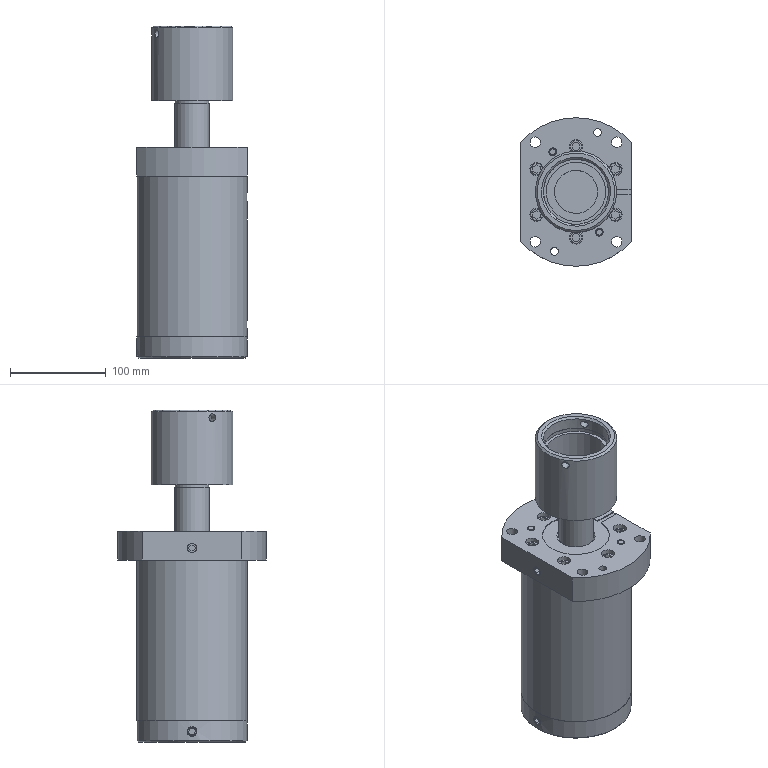Assembly | NX | mm | 25 component files | 25 solids | 539 faces | box 115 x 155 x 346.63 mm | volume 2246698 mm3 | plane 236 | cylinder 227 | cone 66 | spline 10 | commonest cylinder face diameters 1 x84 8 x24 7 x14 9 x12 14 x12 7.785 x12 13 x12 75 x9
Bill of materials:
unnamed part 1 | 2 |  | Solid short cylinder with chamfered edges at both ends; length roughly equal to diameter.
unnamed part 2 | 1 |  | Stepped rotational part: a large hollow cylindrical cup head on a long, narrower shaft that steps down to smaller diameters at the far end.
unnamed part 3 | 1 |  | Thin flat annular ring with a rectangular cross-section.
unnamed part 4 | 12 |  | Headed fastener-like part: a cylindrical head with a hexagonal socket recess on a plain cylindrical shank with a chamfered tip.
unnamed part 5 | 1 |  | Thick-walled cylindrical sleeve or tube with a ring of axial holes in the end face and radial holes in the side wall.
unnamed part 6 | 1 |  | Cylindrical body with a central through bore and a raised annular boss on top; the outer surface has several evenly spaced circumferential lines, as if made of stacked discs.
unnamed part 7 | 1 |  | Hexagonal nut-like body with a plain central through bore and chamfered corners on both faces.
unnamed part 8 | 1 |  | Helical coil spring with about 11 to 12 open coils; the end coils appear closed and flattened.
unnamed part 9 | 1 |  | Helical coil spring with about 11 to 12 open coils and a flat-faced end coil, nearly identical in shape to the other coil spring in this set.
unnamed part 10 | 1 |  | Circular flat disc or flange with a bolt circle of six through holes, plus two smaller holes and a shallow arc-shaped feature on the top face.
unnamed part 11 | 2 |  | Slender solid cylindrical pin with chamfered ends.
unnamed part 12 | 1 |  | Thick plate with two parallel straight sides and two arc-shaped ends, a central stepped bore, many holes through the plate, and a short cylindrical spigot on the underside.
Mates:
1. fix | cylinder_body 1 component
2. concentric | cylinder_body 1 edge | rear_cover 1 edge
3. distance | rear_cover 1 face | cylinder_body 1 face
4. concentric | front_cover 1 edge | cylinder_body 1 edge
5. parallel | front_cover 1 face | rear_cover 1 face
6. concentric | piston 1 edge | piston_rod 1 edge
7. touch align | piston_rod 1 face | front_cover 1 face
8. concentric | screw_plug 2 edge | front_cover 1 edge
9. touch align | SPRING_CYLINDER_COMPRESSION_1 2 datumaxis | screw_plug 2 face
10. touch align | SPRING_CYLINDER_COMPRESSION_1 2 face | screw_plug 2 face
11. touch align | SPRING_CYLINDER_COMPRESSION_1 1 datumaxis | screw_plug 1 face
12. touch align | SPRING_CYLINDER_COMPRESSION_1 1 face | screw_plug 1 face
13. touch align | screw_plug 1 face | rear_cover 1 face
14. touch align | screw_plug 1 face | rear_cover 1 face
15. concentric | O_ring 1 arc | front_cover 1 edge
16. concentric | pin 2 edge | front_cover 1 edge
17. concentric | pin 1 edge | front_cover 1 edge
18. concentric | screw_M8X30 12 edge | front_cover 1 edge
19. parallel | screw_M8X30 12 face | front_cover 1 face
20. fix | assembly component
21. bond | screw_M8X30 12 component | assembly component
22. bond | screw_M8X30 11 component | assembly component
23. bond | screw_M8X30 10 component | assembly component
24. bond | screw_M8X30 9 component | assembly component
25. circular | assembly datumaxis | assembly cartesiancoordinatesystem | assembly cartesiancoordinatesystem | assembly cartesiancoordinatesystem | assembly cartesiancoordinatesystem | assembly cartesiancoordinatesystem | assembly cartesiancoordinatesystem
26. bond | screw_M8X30 8 component | assembly component
27. bond | screw_M8X30 7 component | assembly component
28. concentric | screw_M8X30 6 edge | rear_cover 1 edge
29. parallel | screw_M8X30 6 face | front_cover 1 edge
30. fix | assembly component
31. bond | screw_M8X30 6 component | assembly component
32. bond | screw_M8X30 5 component | assembly component
33. bond | screw_M8X30 4 component | assembly component
34. bond | screw_M8X30 3 component | assembly component
35. bond | screw_M8X30 2 component | assembly component
36. bond | screw_M8X30 1 component | assembly component
37. circular | assembly datumaxis | assembly cartesiancoordinatesystem | assembly cartesiancoordinatesystem | assembly cartesiancoordinatesystem | assembly cartesiancoordinatesystem | assembly cartesiancoordinatesystem | assembly cartesiancoordinatesystem
38. concentric | nut_M27 1 edge | piston 1 edge
39. parallel | nut_M27 1 face | front_cover 1 face